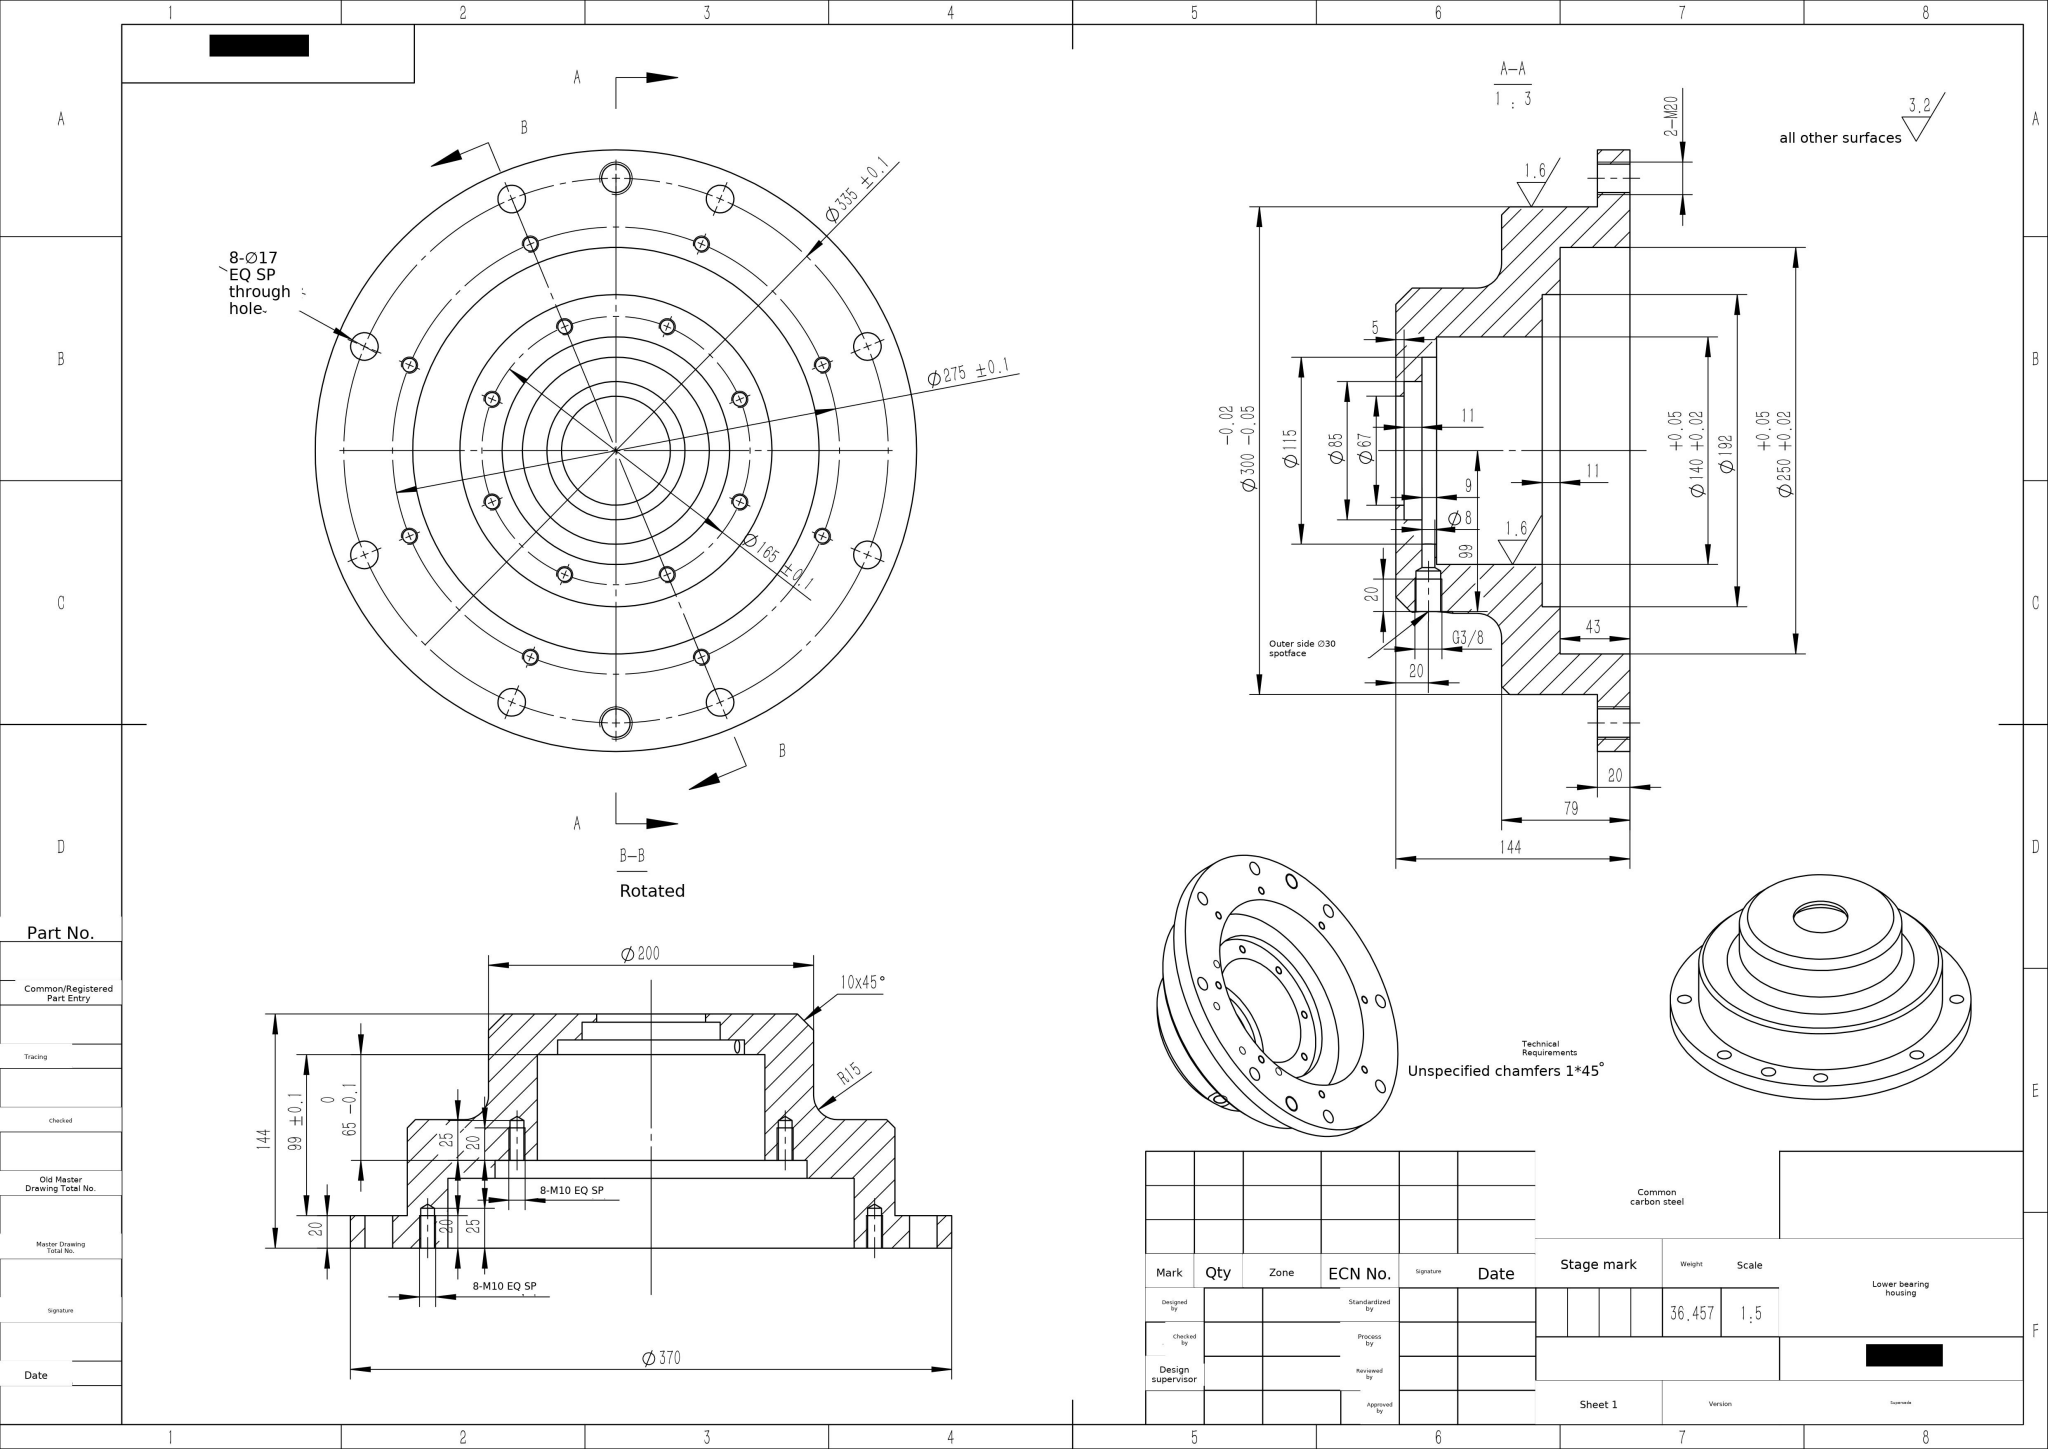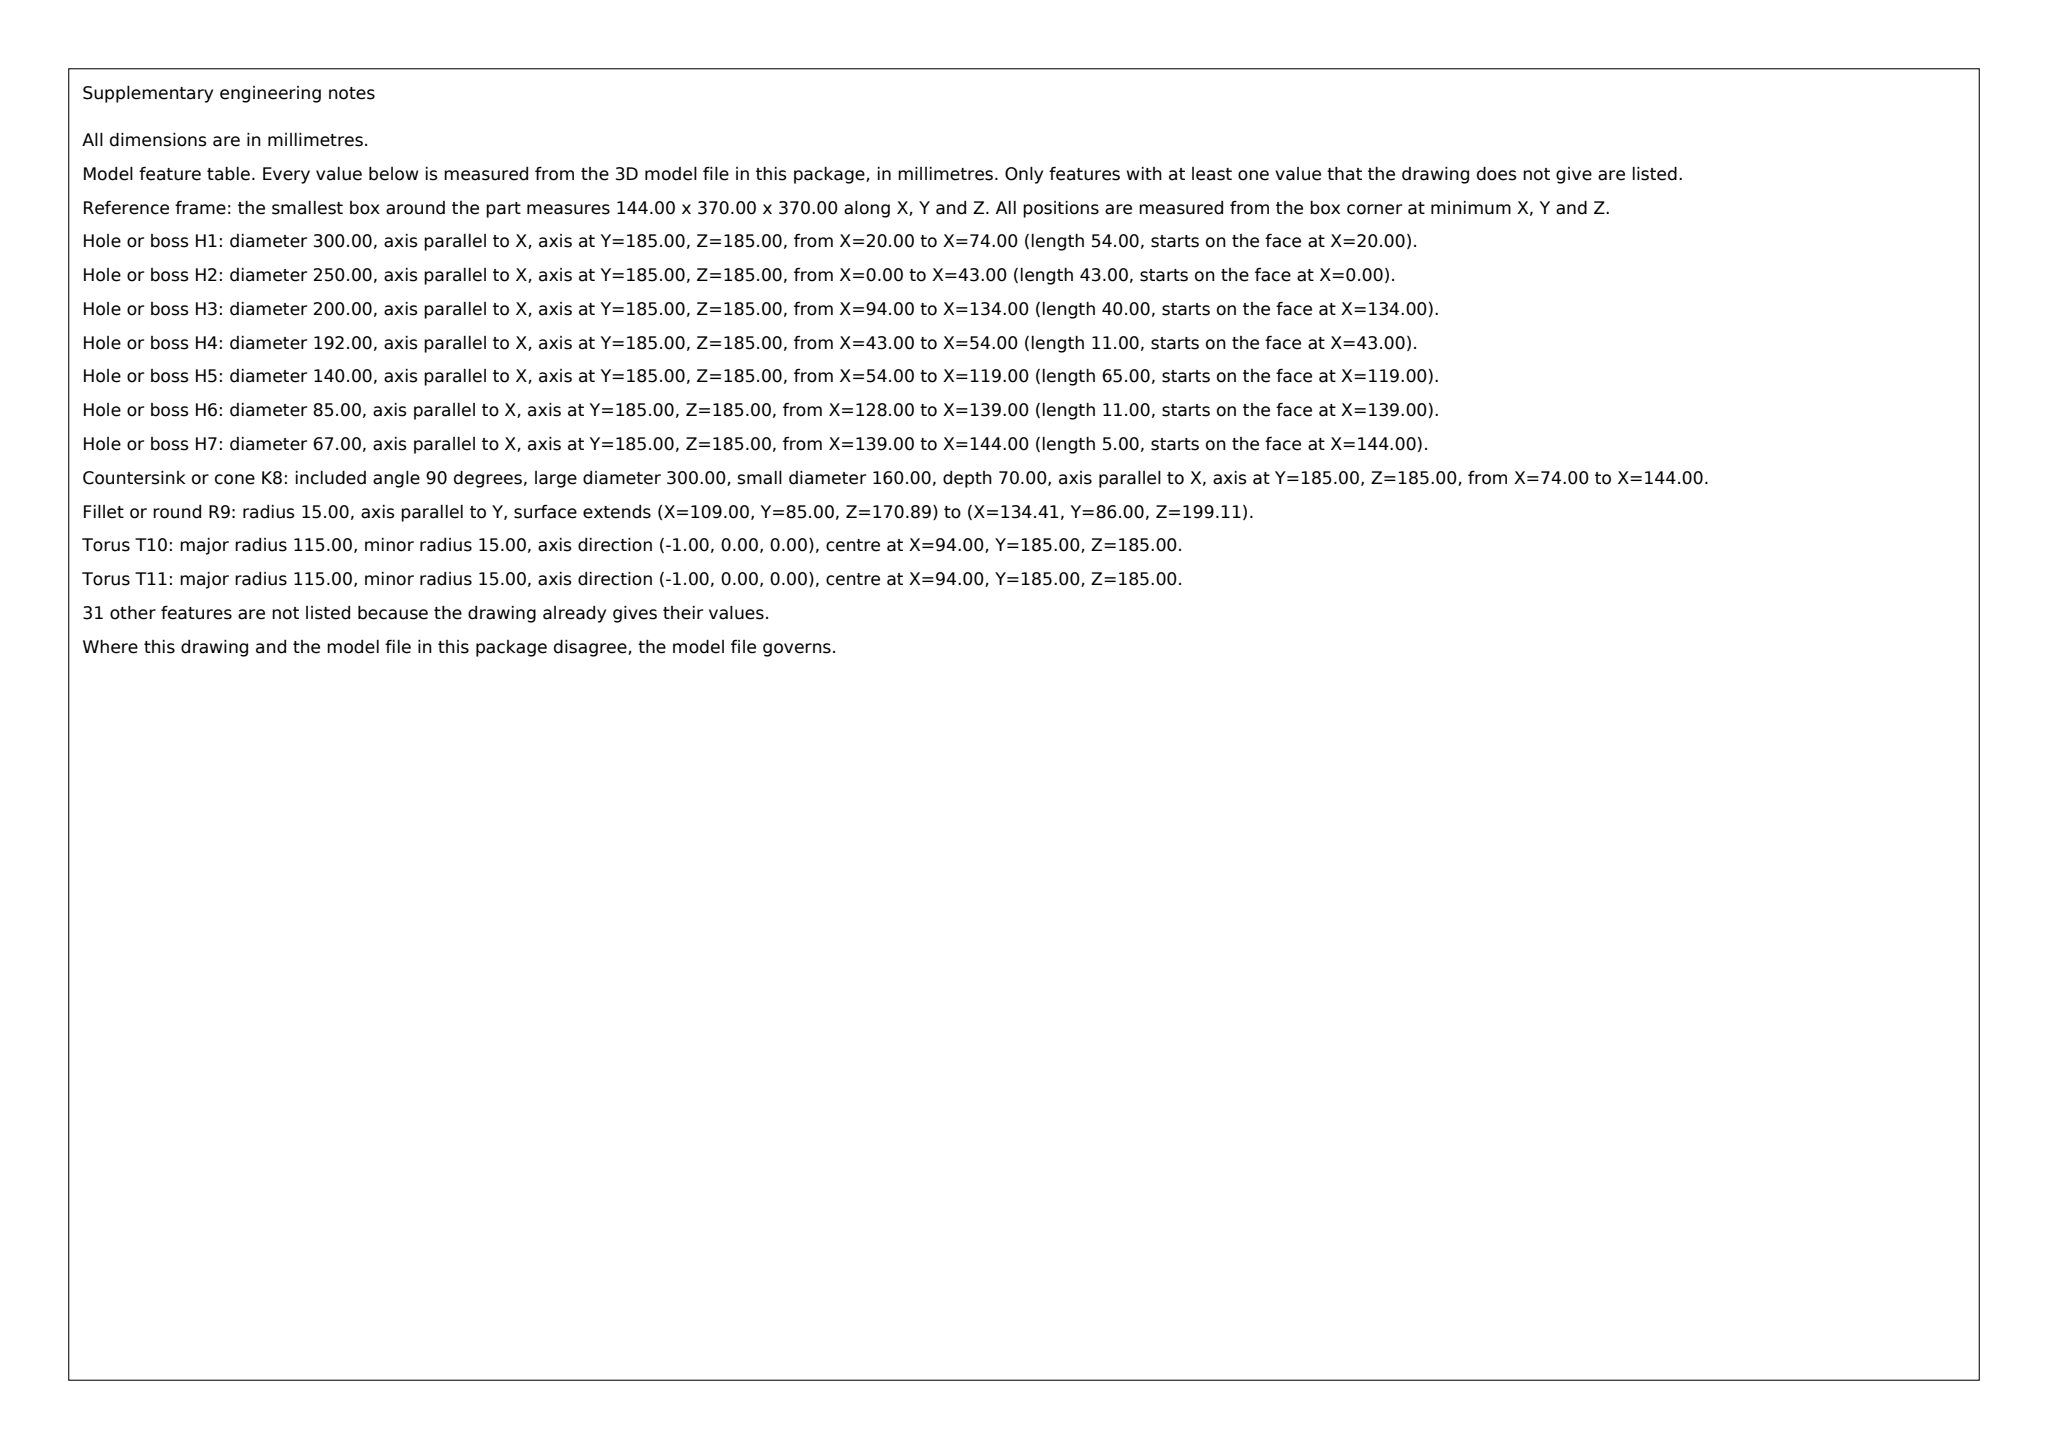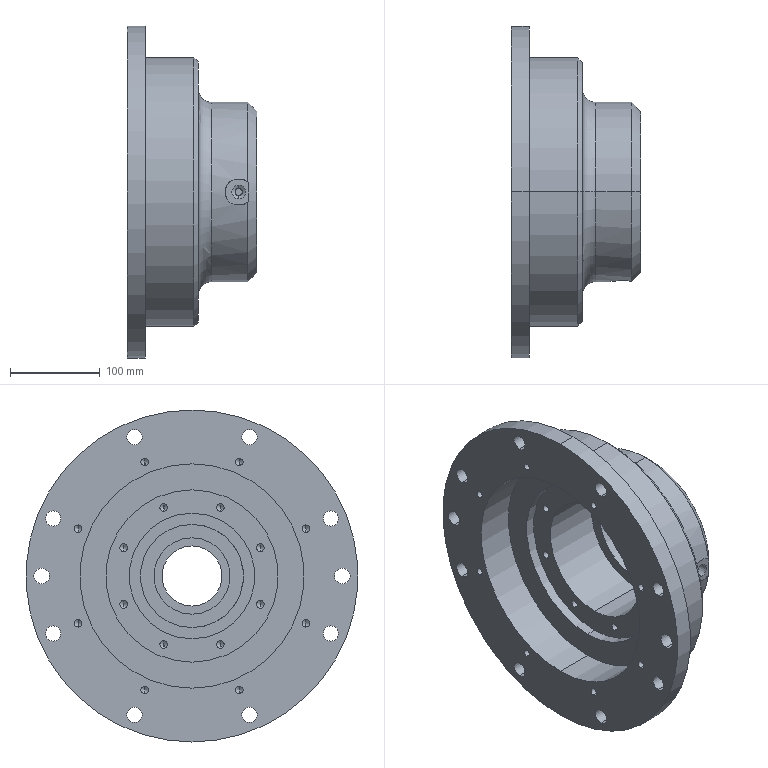Part | SolidWorks | mm | material Common carbon steel | 1 solid | 127 faces | box 144 x 370 x 370 mm | volume 4673963 mm3 | cylinder 77 | cone 38 | plane 10 | torus 2 | commonest cylinder face diameters 8.5 x32 17 x16 17.5 x4 30 x3 15.25 x2 8 x2 192 x2 140 x2
build123d program:
from build123d import *

# Parameters (mm, degrees)
CHAMFER1_SIZE           = 10
CUT_EXTRUDE1_REACH      = 300.64
SKETCH3_R               = 8.5
CIRPATTERN1_COUNT       = 8
CIRPATTERN2_COUNT       = 8
CIRPATTERN3_COUNT       = 8
FILLET1_R               = 15
CHAMFER2_SIZE           = 5
M20_TAPPED_HOLE1_D      = 17.5
CIRPATTERN4_COUNT       = 2
SKETCH10_R              = 4
CUT_EXTRUDE3_DEPTH      = 80
CUT_EXTRUDE6_START      = -99
SKETCH11_R              = 15
CUT_EXTRUDE6_DEPTH      = 130
G3_8_TAPPED_HOLE1_D     = 15.25
G3_8_TAPPED_HOLE1_DEPTH = 25
G3_8_TAPPED_HOLE1_TIP   = 4.582


with BuildPart() as part:
    # Sketch1 → Revolve1 (revolve)
    with BuildSketch(Plane.XY, mode=Mode.PRIVATE) as revolve1_sk:
        Polygon((0, 125), (0, 185), (20, 185), (20, 150), (79, 150), (79, 100), (144, 100), (144, 33.5), (139, 33.5), (139, 42.5), (128, 42.5), (128, 57.5), (119, 57.5), (119, 70), (54, 70), (54, 96), (43, 96), (43, 125), align=None)
    revolve(revolve1_sk.sketch.rotate(Axis((0, 0, 0), (1, 0, 0)), 90), axis=Axis((0, 0, 0), (1, 0, 0)))

    # Chamfer1
    chamfer1_edges = [part.edges().sort_by_distance(p)[0] for p in [
        (144, 0, -100),
    ]]
    chamfer(chamfer1_edges, length=CHAMFER1_SIZE)

    # Sketch3 → Cut-Extrude1 (cut, up to next)
    with BuildSketch(Plane.ZY, mode=Mode.PRIVATE) as cut_extrude1_sk1:
        with Locations((-64.099, 154.75)):
            Circle(SKETCH3_R)
    cut_extrude1_tool1 = extrude(cut_extrude1_sk1.sketch, amount=-CUT_EXTRUDE1_REACH, mode=Mode.PRIVATE) & part.part
    cut_extrude1 = cut_extrude1_tool1.solids().sort_by_distance((0, 154.75, -64.099))[0]
    add(cut_extrude1, mode=Mode.SUBTRACT)

    # CirPattern1: Cut-Extrude1 ×8 about axis
    cirpattern1_axis = Axis((0, 0, 0), (1, 0, 0))
    for i in range(1, CIRPATTERN1_COUNT):
        add(cut_extrude1.rotate(cirpattern1_axis, i * 360 / CIRPATTERN1_COUNT), mode=Mode.SUBTRACT)

    # Sketch5 → M10 Tapped Hole1 (revolve, cut)
    with BuildSketch(Plane(origin=(0, 127.033, -52.619), x_dir=(0, 0, 1), z_dir=(0, 1, 0))):
        Polygon((0, 0), (0, 27.054), (4.25, 24.5), (4.25, 0), align=None)
    m10_tapped_hole1 = revolve(axis=Axis((-6.35, 127.033, -52.619), (1, 0, 0)), mode=Mode.SUBTRACT)

    # CirPattern2: M10 Tapped Hole1 ×8 about axis
    cirpattern2_axis = Axis((0, 0, 0), (1, 0, 0))
    for i in range(1, CIRPATTERN2_COUNT):
        add(m10_tapped_hole1.rotate(cirpattern2_axis, i * 360 / CIRPATTERN2_COUNT), mode=Mode.SUBTRACT)

    # Sketch7 → M10 Tapped Hole2 (revolve, cut)
    with BuildSketch(Plane(origin=(54, 76.22, -31.571), x_dir=(0, 0, 1), z_dir=(0, 1, 0))):
        Polygon((0, 0), (0, 27.054), (4.25, 24.5), (4.25, 0), align=None)
    m10_tapped_hole2 = revolve(axis=Axis((47.65, 76.22, -31.571), (1, 0, 0)), mode=Mode.SUBTRACT)

    # CirPattern3: M10 Tapped Hole2 ×8 about axis
    cirpattern3_axis = Axis((0, 0, 0), (1, 0, 0))
    for i in range(1, CIRPATTERN3_COUNT):
        add(m10_tapped_hole2.rotate(cirpattern3_axis, i * 360 / CIRPATTERN3_COUNT), mode=Mode.SUBTRACT)

    # Fillet1
    fillet1_edges = [part.edges().sort_by_distance(p)[0] for p in [
        (79, 0, -100),
    ]]
    fillet(fillet1_edges, radius=FILLET1_R)

    # Chamfer2
    chamfer2_edges = [part.edges().sort_by_distance(p)[0] for p in [
        (79, 0, -150),
    ]]
    chamfer(chamfer2_edges, length=CHAMFER2_SIZE)

    # M20 Tapped Hole1 (through all)
    with Locations(Plane(origin=(0, 167.5, 0), x_dir=(0, 0, -1), z_dir=(-1, 0, 0))):
        with Locations((0, 0)):
            m20_tapped_hole1 = Hole(M20_TAPPED_HOLE1_D / 2)

    # CirPattern4: M20 Tapped Hole1 ×2 about axis
    cirpattern4_axis = Axis((0, 0, 0), (1, 0, 0))
    for i in range(1, CIRPATTERN4_COUNT):
        add(m20_tapped_hole1.rotate(cirpattern4_axis, i * 360 / CIRPATTERN4_COUNT), mode=Mode.SUBTRACT)

    # Sketch10 → Cut-Extrude3 (cut)
    with BuildSketch(Plane(origin=(0, 0, 0), x_dir=(1, 0, 0), z_dir=(0, 1, 0))):
        with Locations(Location((124, 0, 0), (0, 0, 270))):
            Circle(SKETCH10_R)
    extrude(amount=-CUT_EXTRUDE3_DEPTH, mode=Mode.SUBTRACT)

    # Sketch11 → Cut-Extrude6 (cut)
    with BuildSketch(Plane(origin=(0, 0, 0), x_dir=(1, 0, 0), z_dir=(0, 1, 0)).offset(CUT_EXTRUDE6_START)):
        with Locations((124, 0)):
            Circle(SKETCH11_R)
    extrude(amount=-CUT_EXTRUDE6_DEPTH, mode=Mode.SUBTRACT)

    # G3_8 Tapped Hole1
    with Locations(Plane(origin=(124, -99, 0), x_dir=(0, 0, -1), z_dir=(0, -1, 0))):
        with Locations((0, 0)):
            Hole(G3_8_TAPPED_HOLE1_D / 2, depth=G3_8_TAPPED_HOLE1_DEPTH)
            with Locations((0, 0, -(G3_8_TAPPED_HOLE1_DEPTH + G3_8_TAPPED_HOLE1_TIP / 2))):  # 118° drill point
                Cone(0, G3_8_TAPPED_HOLE1_D / 2, G3_8_TAPPED_HOLE1_TIP, mode=Mode.SUBTRACT)


solid = part.part